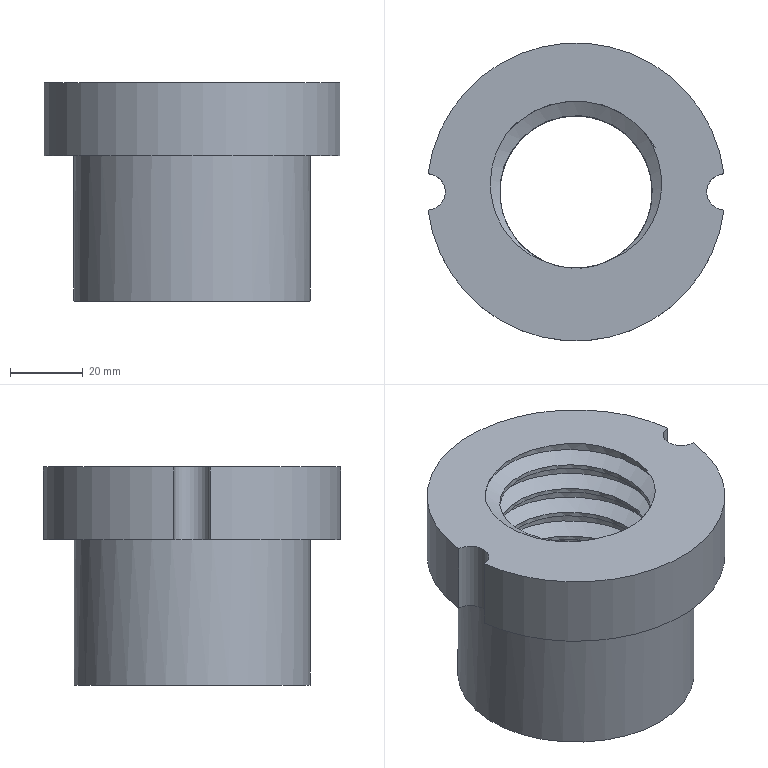Component | NX | SCREW_SLEEVE | 1 solid | 14 faces | volume 132149 mm3 | cylinder 8 | plane 4 | spline 2 | commonest cylinder face diameters 82 x2 10 x2 42 x1 65 x1 50 x1 50.5 x1